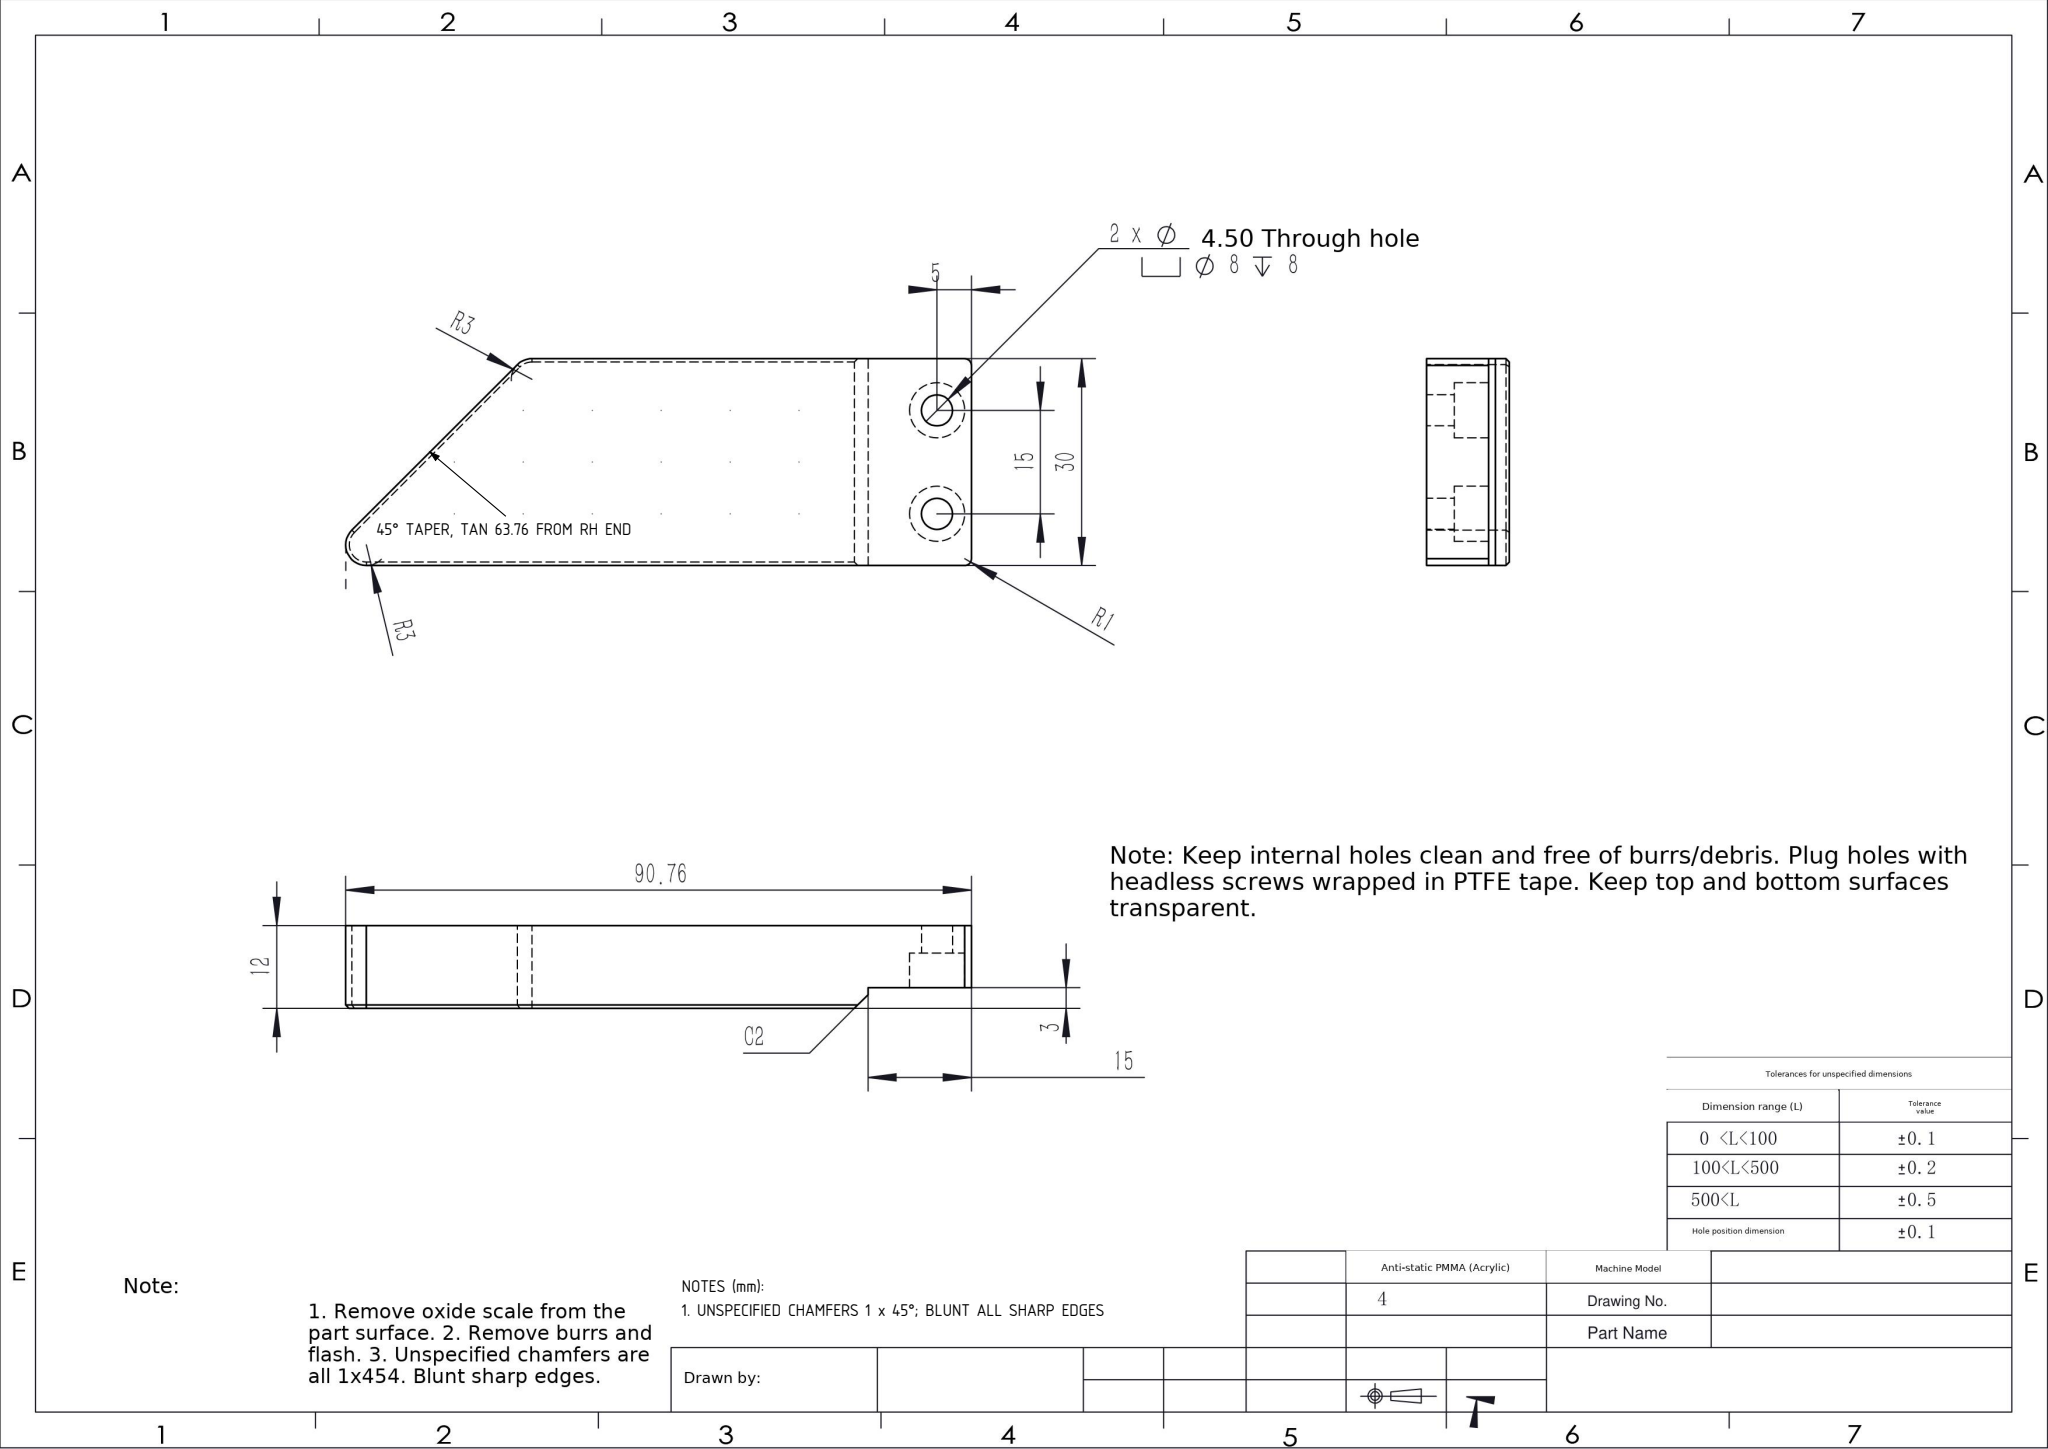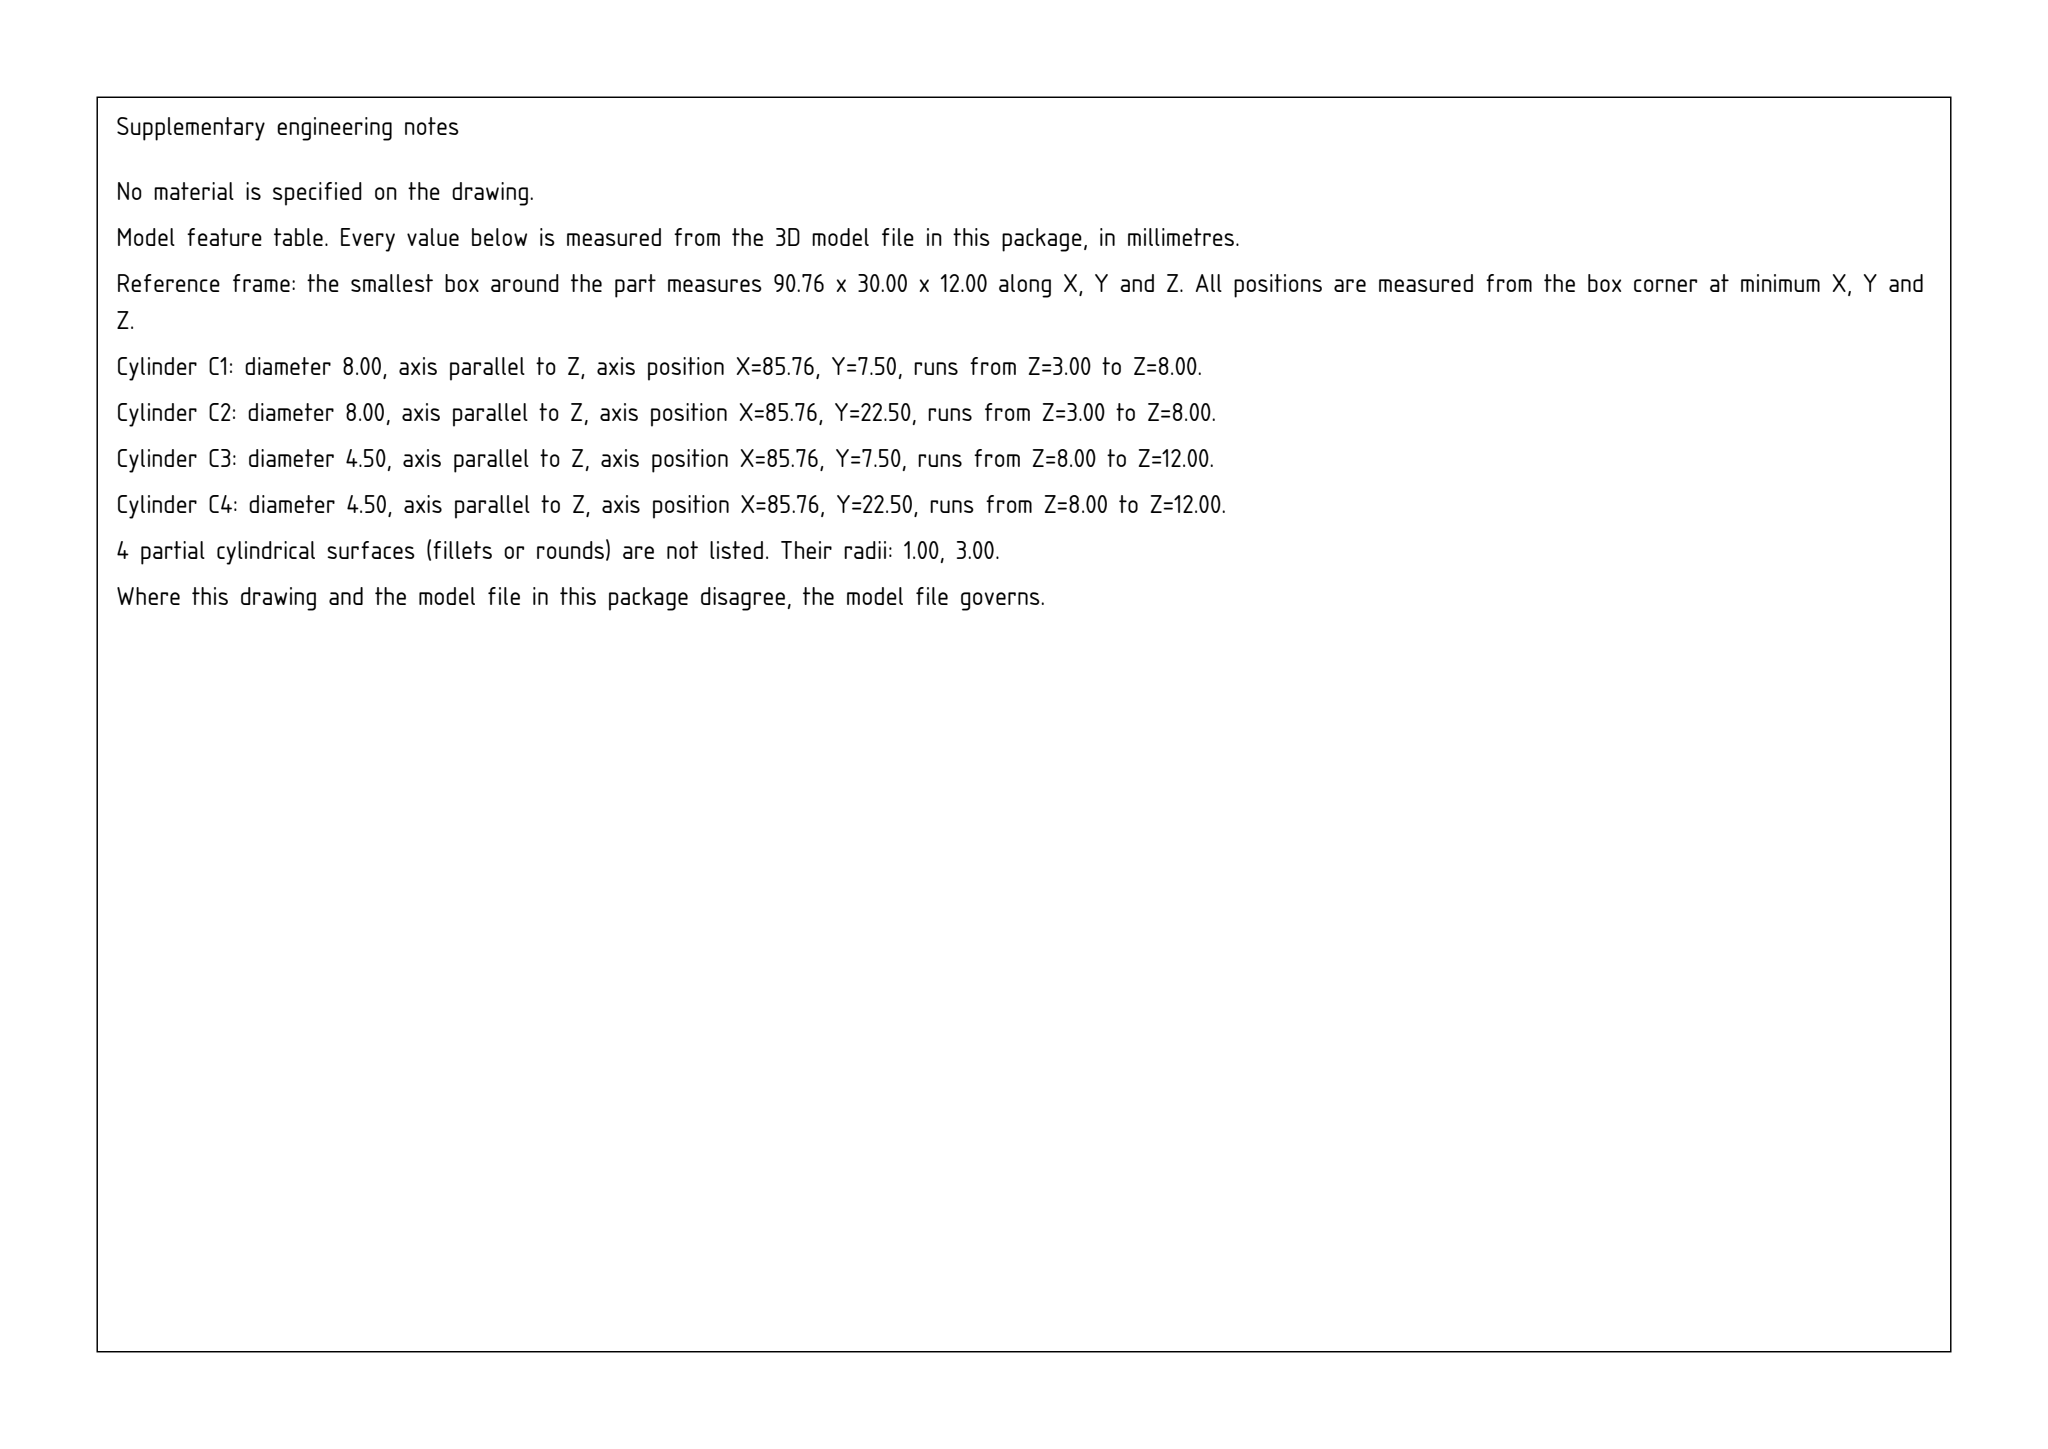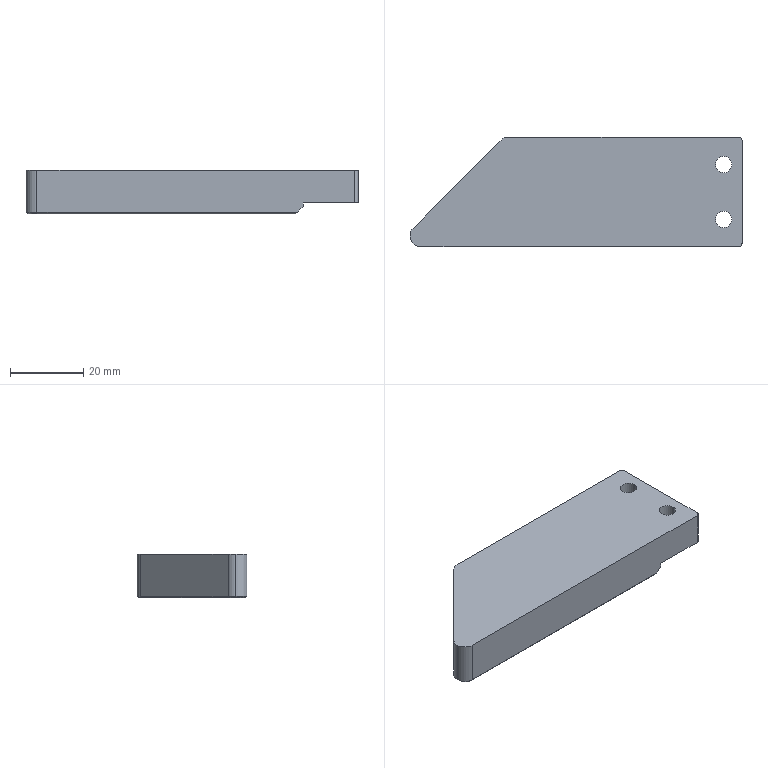Part | SolidWorks | mm | material Anti-static PMMA (Acrylic) | 1 solid | 29 faces | box 90.76 x 30 x 12 mm | volume 26600 mm3 | plane 14 | cylinder 13 | cone 2 | commonest cylinder face diameters 8 x4 4.5 x4 6 x3 2 x2
Drawing notes:
TAPERED LEFT END: 45° DIAG, TANGENT 63.76 FROM RIGHT END FACE | from the solid: 45° edge tangent to R3 fillets at (3,3) & (27,27); tangency on Y=30 top edge at X=27, i.e. 90.76-27=63.76 from X=90.76 end plane
UNSPECIFIED CHAMFERS 1 x 45°; BLUNT ALL SHARP EDGES | from the solid: inclined_planes list angle_to_xyz_axes 45/45/90 and 90/45/45 (45° chamfer faces, e.g. 2x2 C2 at x=73.8 and 0.5 edge breaks)
build123d program:
from build123d import *

# Parameters (mm, degrees)
SKETCH1_W                                            = 95
SKETCH1_H                                            = 30
BOSS_EXTRUDE1_DEPTH                                  = 12
HOLE_SIZE_ACCORDING_TO_THE_TYPE_OF_HEXAG_D           = 4.5
HOLE_SIZE_ACCORDING_TO_THE_TYPE_OF_HEXAG_CBORE_D     = 8
HOLE_SIZE_ACCORDING_TO_THE_TYPE_OF_HEXAG_CBORE_DEPTH = 8
SKETCH4_W                                            = 15
SKETCH4_H                                            = 30
CUT_EXTRUDE1_DEPTH                                   = 3
SKETCH5_R                                            = 2
BOSS_EXTRUDE2_DEPTH                                  = 76
FILLET2_R                                            = 1
CUT_EXTRUDE5_DEPTH                                   = 52.237
CUT_EXTRUDE5_DEPTH_BACK                              = 52.237
FILLET3_R                                            = 3
CHAMFER1_SIZE                                        = 2
CHAMFER2_SIZE                                        = 0.5


with BuildPart() as part:
    # Sketch1 → Boss-Extrude1 (new body)
    with BuildSketch(Plane.XY):
        Rectangle(SKETCH1_W, SKETCH1_H)
    extrude(amount=BOSS_EXTRUDE1_DEPTH)

    # Hole size according to the type of hexag (through all)
    with Locations(Plane(origin=(0, 0, 0), x_dir=(-1, 0, 0), z_dir=(0, 0, -1))):
        with Locations((-42.5, -7.5), (-42.5, 7.5)):
            CounterBoreHole(HOLE_SIZE_ACCORDING_TO_THE_TYPE_OF_HEXAG_D / 2, HOLE_SIZE_ACCORDING_TO_THE_TYPE_OF_HEXAG_CBORE_D / 2, HOLE_SIZE_ACCORDING_TO_THE_TYPE_OF_HEXAG_CBORE_DEPTH)

    # Sketch4 → Cut-Extrude1 (cut)
    with BuildSketch(Plane(origin=(0, 0, 0), x_dir=(-1, 0, 0), z_dir=(0, 0, -1))):
        with Locations((-40, 0)):
            Rectangle(SKETCH4_W, SKETCH4_H)
    extrude(amount=-CUT_EXTRUDE1_DEPTH, mode=Mode.SUBTRACT)

    # Sketch5 → Boss-Extrude2 (add)
    with BuildSketch(Plane.ZY.offset(47.5)):
        with Locations((6, 0)):
            Circle(SKETCH5_R)
    extrude(amount=-BOSS_EXTRUDE2_DEPTH)

    # Fillet2
    fillet2_edges = [part.edges().sort_by_distance(p)[0] for p in [
        (47.5, -15, 7.5),
        (47.5, 15, 7.5),
    ]]
    fillet(fillet2_edges, radius=FILLET2_R)

    # Sketch9 → Cut-Extrude5 (cut, two sides: drawn at the far end of the back side and taken through both)
    with BuildSketch(Plane(origin=(0, 0, 0), x_dir=(-1, 0, 0), z_dir=(0, 0, -1)).offset(-CUT_EXTRUDE5_DEPTH_BACK)):
        Polygon((195.461, -162.961), (47.5, -15), (17.5, 15), (-130.461, 162.961), (165.461, 458.883), (491.383, 132.961), align=None)
    extrude(amount=CUT_EXTRUDE5_DEPTH + CUT_EXTRUDE5_DEPTH_BACK, mode=Mode.SUBTRACT)

    # Fillet3
    fillet3_edges = [part.edges().sort_by_distance(p)[0] for p in [
        (-17.5, 15, 6),
        (-47.5, -15, 6),
    ]]
    fillet(fillet3_edges, radius=FILLET3_R)

    # Chamfer1
    chamfer1_edges = [part.edges().sort_by_distance(p)[0] for p in [
        (32.5, 0, 0),
    ]]
    chamfer(chamfer1_edges, length=CHAMFER1_SIZE)

    # Chamfer2
    chamfer2_edges = [part.edges().sort_by_distance(p)[0] for p in [
        (-4.879, -15, 0),
        (-30.379, 2.121, 0),
        (-17.405, 14.772, 0),
        (-43.029, -13.148, 0),
        (7.121, 15, 0),
    ]]
    chamfer(chamfer2_edges, length=CHAMFER2_SIZE)


solid = part.part